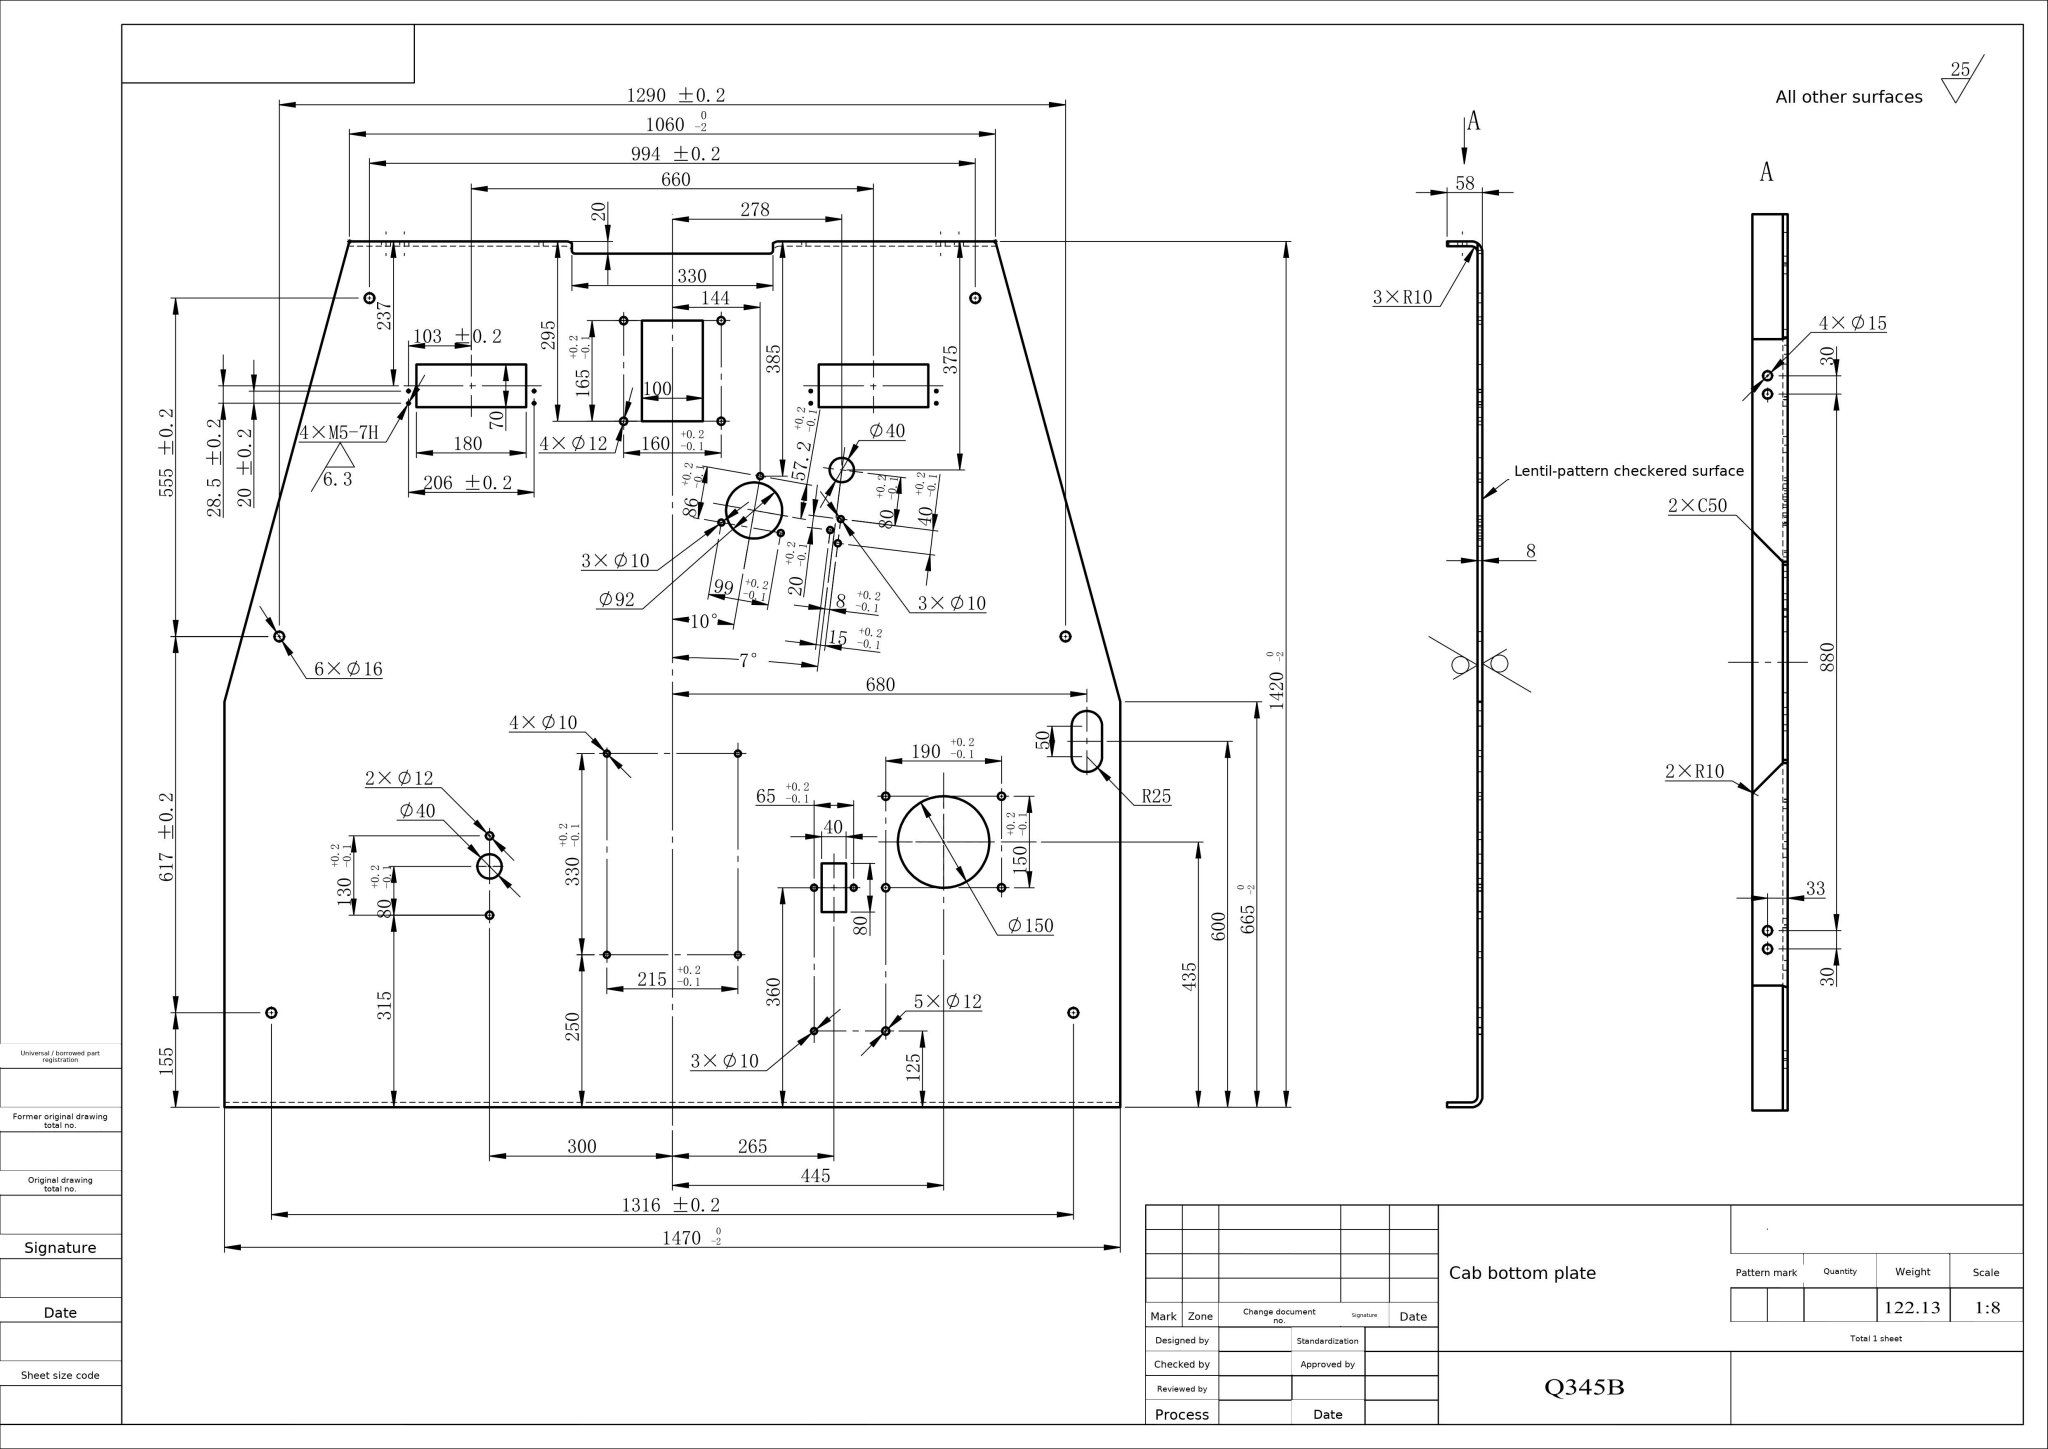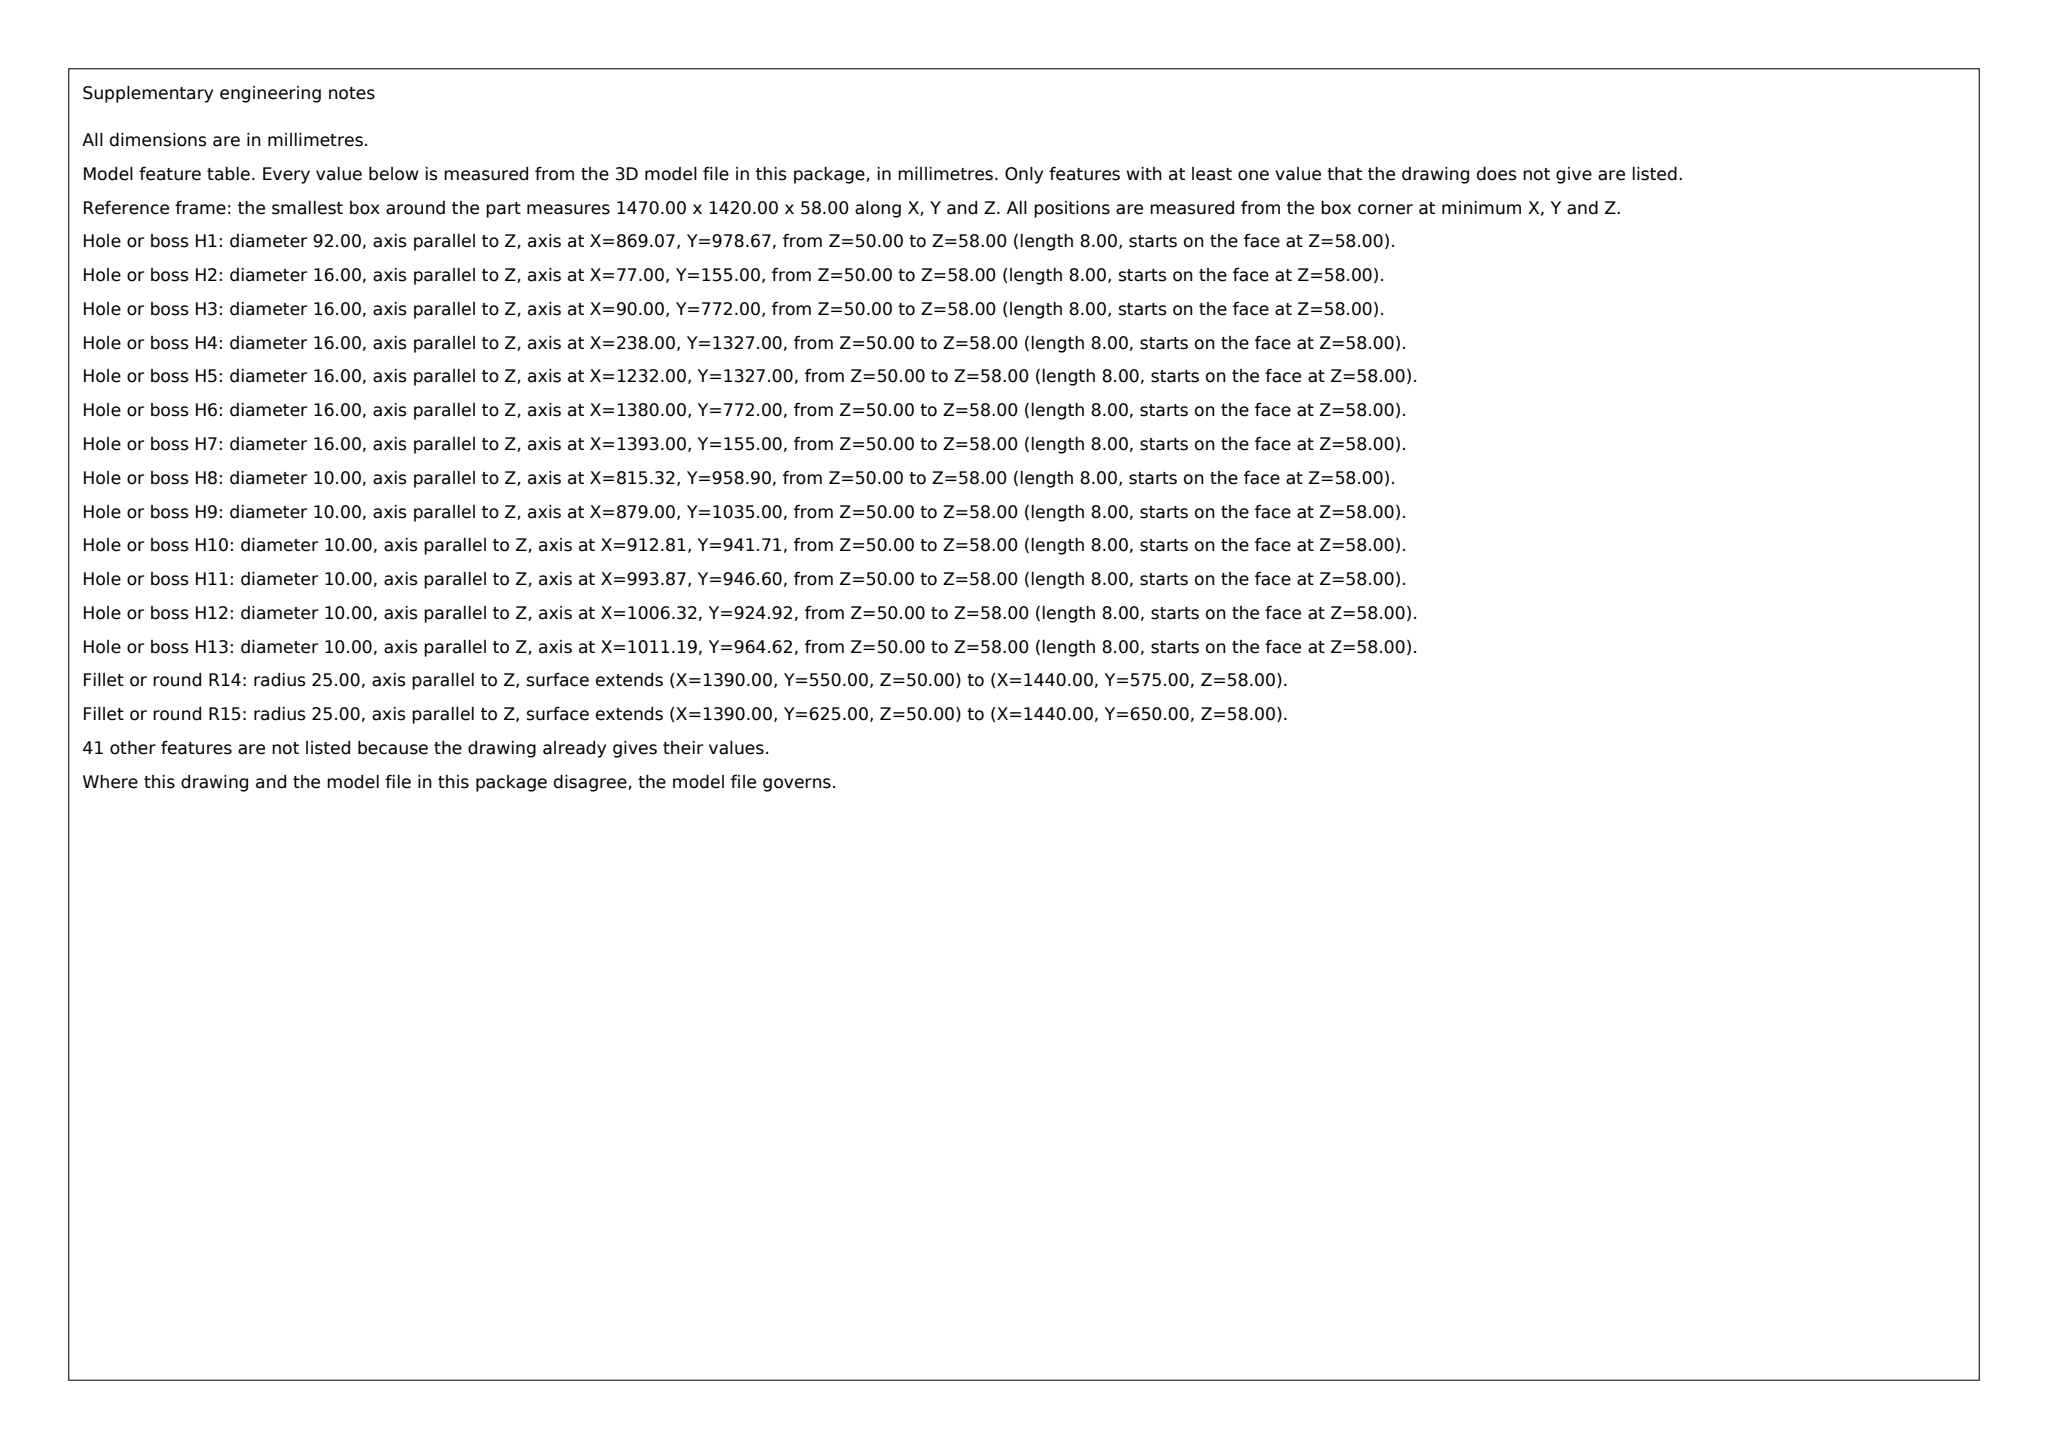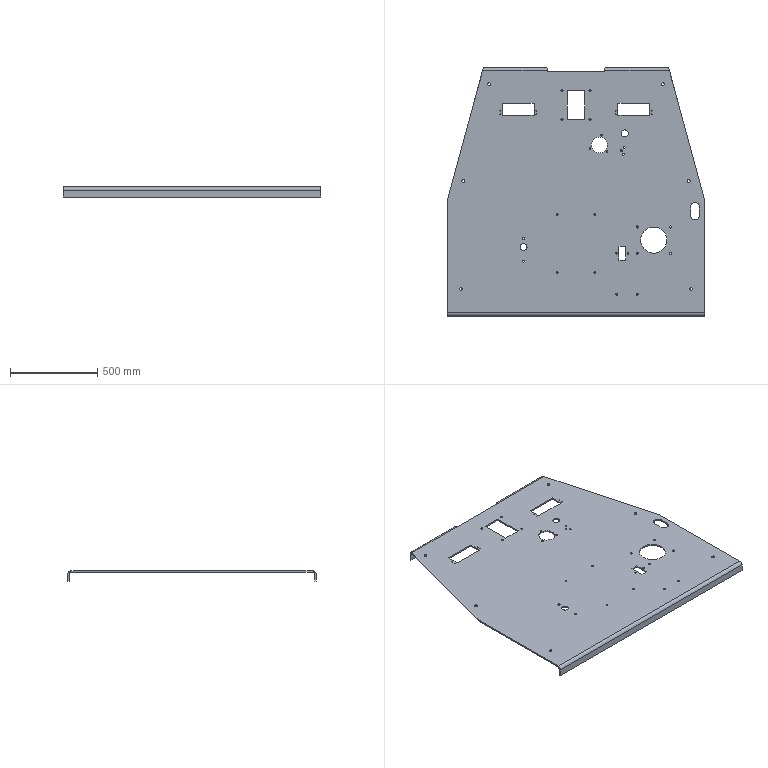Part | SolidWorks | mm | material Q345B | 1 solid | 144 faces | box 1470 x 1420 x 58 mm | volume 15518421 mm3 | cylinder 104 | plane 40 | commonest cylinder face diameters 10 x28 12 x22 4.2 x16 16 x12 15 x8 20 x5 40 x4 36 x3